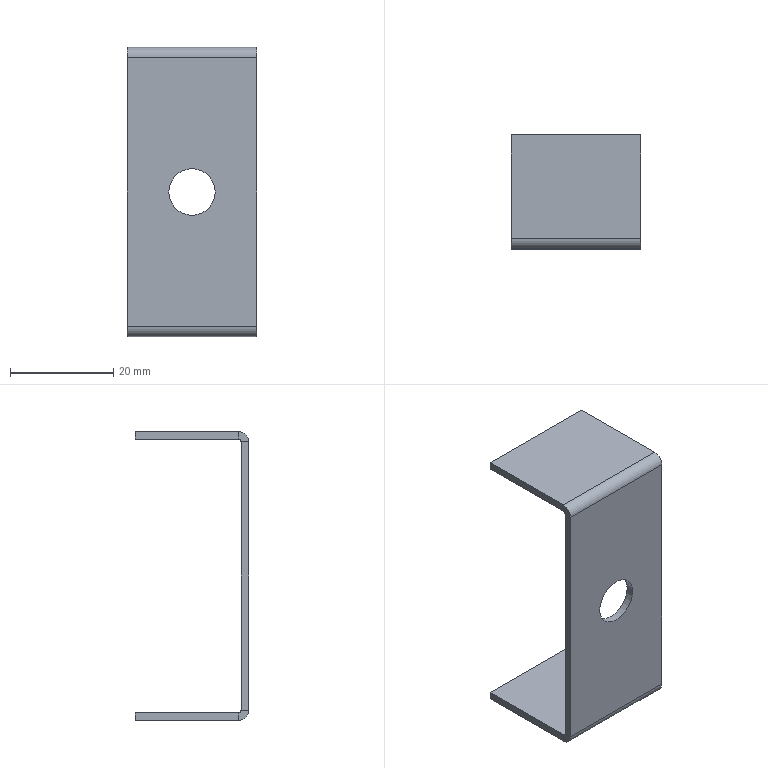Component | SolidWorks | BrowBracketAssembly3-1_BrowBracket-1 | 1 solid | 24 faces | box 25 x 22 x 56 mm | volume 3502 mm3 | plane 18 | cylinder 6 | commonest cylinder face diameters 9 x2 4 x2 1 x2
STEP:
#1=COLOUR_RGB('',0.7922,0.8196,0.9333);
#2=FILL_AREA_STYLE_COLOUR('',#1);
#3=FILL_AREA_STYLE('',(#2));
#4=SURFACE_STYLE_FILL_AREA(#3);
#5=SURFACE_SIDE_STYLE('',(#4));
#6=SURFACE_STYLE_USAGE(.BOTH.,#5);
#7=PRESENTATION_STYLE_ASSIGNMENT((#6));
#8=CARTESIAN_POINT('',(-2.047,6.292,1.181));
#9=VERTEX_POINT('',#8);
#10=CARTESIAN_POINT('',(-1.693,6.292,1.181));
#11=VERTEX_POINT('',#10);
#12=CARTESIAN_POINT('',(-1.87,6.292,1.181));
#13=DIRECTION('',(-0.,-1.,-0.));
#14=DIRECTION('',(1.,-0.,0.));
#15=AXIS2_PLACEMENT_3D('',#12,#13,#14);
#16=CIRCLE('',#15,0.1772);
#17=EDGE_CURVE('',#9,#11,#16,.T.);
#18=ORIENTED_EDGE('',*,*,#17,.F.);
#19=CARTESIAN_POINT('',(-2.047,6.233,1.181));
#20=VERTEX_POINT('',#19);
#21=CARTESIAN_POINT('',(-2.047,6.292,1.181));
#22=DIRECTION('',(-0.,-1.,-0.));
#23=VECTOR('',#22,39.37);
#24=LINE('',#21,#23);
#25=EDGE_CURVE('',#9,#20,#24,.T.);
#26=ORIENTED_EDGE('',*,*,#25,.T.);
#27=CARTESIAN_POINT('',(-1.693,6.233,1.181));
#28=VERTEX_POINT('',#27);
#29=CARTESIAN_POINT('',(-1.87,6.233,1.181));
#30=DIRECTION('',(-0.,-1.,-0.));
#31=DIRECTION('',(1.,-0.,0.));
#32=AXIS2_PLACEMENT_3D('',#29,#30,#31);
#33=CIRCLE('',#32,0.1772);
#34=EDGE_CURVE('',#20,#28,#33,.T.);
#35=ORIENTED_EDGE('',*,*,#34,.T.);
#36=CARTESIAN_POINT('',(-1.693,6.292,1.181));
#37=DIRECTION('',(-0.,-1.,-0.));
#38=VECTOR('',#37,39.37);
#39=LINE('',#36,#38);
#40=EDGE_CURVE('',#11,#28,#39,.T.);
#41=ORIENTED_EDGE('',*,*,#40,.F.);
#42=EDGE_LOOP('',(#18,#26,#35,#41));
#43=FACE_OUTER_BOUND('',#42,.T.);
#44=CARTESIAN_POINT('',(-1.87,6.292,1.181));
#45=DIRECTION('',(-0.,-1.,-0.));
#46=DIRECTION('',(1.,-0.,0.));
#47=AXIS2_PLACEMENT_3D('',#44,#45,#46);
#48=CYLINDRICAL_SURFACE('',#47,0.1772);
#49=ADVANCED_FACE('',(#43),#48,.F.);
#50=CARTESIAN_POINT('',(-2.362,6.233,2.204));
#51=VERTEX_POINT('',#50);
#52=CARTESIAN_POINT('',(-2.362,6.292,2.204));
#53=VERTEX_POINT('',#52);
#54=CARTESIAN_POINT('',(-2.362,6.233,2.204));
#55=DIRECTION('',(0.,1.,0.));
#56=VECTOR('',#55,39.37);
#57=LINE('',#54,#56);
#58=EDGE_CURVE('',#51,#53,#57,.T.);
#59=ORIENTED_EDGE('',*,*,#58,.F.);
#60=CARTESIAN_POINT('',(-2.362,6.311,2.283));
#61=VERTEX_POINT('',#60);
#62=CARTESIAN_POINT('',(-2.362,6.311,2.204));
#63=DIRECTION('',(1.,-0.,0.));
#64=DIRECTION('',(-0.,-1.,-0.));
#65=AXIS2_PLACEMENT_3D('',#62,#63,#64);
#66=CIRCLE('',#65,0.07874);
#67=EDGE_CURVE('',#61,#51,#66,.T.);
#68=ORIENTED_EDGE('',*,*,#67,.F.);
#69=CARTESIAN_POINT('',(-2.362,6.311,2.224));
#70=VERTEX_POINT('',#69);
#71=CARTESIAN_POINT('',(-2.362,6.311,2.224));
#72=DIRECTION('',(-0.,-0.,1.));
#73=VECTOR('',#72,39.37);
#74=LINE('',#71,#73);
#75=EDGE_CURVE('',#70,#61,#74,.T.);
#76=ORIENTED_EDGE('',*,*,#75,.F.);
#77=CARTESIAN_POINT('',(-2.362,6.311,2.204));
#78=DIRECTION('',(1.,-0.,0.));
#79=DIRECTION('',(-0.,-1.,-0.));
#80=AXIS2_PLACEMENT_3D('',#77,#78,#79);
#81=CIRCLE('',#80,0.01969);
#82=EDGE_CURVE('',#70,#53,#81,.T.);
#83=ORIENTED_EDGE('',*,*,#82,.T.);
#84=EDGE_LOOP('',(#59,#68,#76,#83));
#85=FACE_OUTER_BOUND('',#84,.T.);
#86=CARTESIAN_POINT('',(-2.362,6.233,2.204));
#87=DIRECTION('',(-1.,0.,-0.));
#88=DIRECTION('',(-0.,-1.,-0.));
#89=AXIS2_PLACEMENT_3D('',#86,#87,#88);
#90=PLANE('',#89);
#91=ADVANCED_FACE('',(#85),#90,.T.);
#92=CARTESIAN_POINT('',(-2.362,6.233,0.1571));
#93=VERTEX_POINT('',#92);
#94=CARTESIAN_POINT('',(-2.362,6.233,2.283));
#95=DIRECTION('',(0.,0.,-1.));
#96=VECTOR('',#95,39.37);
#97=LINE('',#94,#96);
#98=EDGE_CURVE('',#51,#93,#97,.T.);
#99=ORIENTED_EDGE('',*,*,#98,.F.);
#100=ORIENTED_EDGE('',*,*,#58,.T.);
#101=CARTESIAN_POINT('',(-2.362,6.292,0.1571));
#102=VERTEX_POINT('',#101);
#103=CARTESIAN_POINT('',(-2.362,6.292,2.283));
#104=DIRECTION('',(0.,0.,-1.));
#105=VECTOR('',#104,39.37);
#106=LINE('',#103,#105);
#107=EDGE_CURVE('',#53,#102,#106,.T.);
#108=ORIENTED_EDGE('',*,*,#107,.T.);
#109=CARTESIAN_POINT('',(-2.362,6.292,0.1571));
#110=DIRECTION('',(-0.,-1.,-0.));
#111=VECTOR('',#110,39.37);
#112=LINE('',#109,#111);
#113=EDGE_CURVE('',#102,#93,#112,.T.);
#114=ORIENTED_EDGE('',*,*,#113,.T.);
#115=EDGE_LOOP('',(#99,#100,#108,#114));
#116=FACE_OUTER_BOUND('',#115,.T.);
#117=CARTESIAN_POINT('',(-2.362,6.311,2.224));
#118=DIRECTION('',(-1.,0.,-0.));
#119=DIRECTION('',(-0.,-1.,-0.));
#120=AXIS2_PLACEMENT_3D('',#117,#118,#119);
#121=PLANE('',#120);
#122=ADVANCED_FACE('',(#116),#121,.T.);
#123=CARTESIAN_POINT('',(-1.378,6.311,2.283));
#124=VERTEX_POINT('',#123);
#125=CARTESIAN_POINT('',(-1.378,6.311,2.224));
#126=VERTEX_POINT('',#125);
#127=CARTESIAN_POINT('',(-1.378,6.311,2.283));
#128=DIRECTION('',(0.,0.,-1.));
#129=VECTOR('',#128,39.37);
#130=LINE('',#127,#129);
#131=EDGE_CURVE('',#124,#126,#130,.T.);
#132=ORIENTED_EDGE('',*,*,#131,.F.);
#133=CARTESIAN_POINT('',(-1.378,6.233,2.204));
#134=VERTEX_POINT('',#133);
#135=CARTESIAN_POINT('',(-1.378,6.311,2.204));
#136=DIRECTION('',(1.,-0.,0.));
#137=DIRECTION('',(-0.,-1.,-0.));
#138=AXIS2_PLACEMENT_3D('',#135,#136,#137);
#139=CIRCLE('',#138,0.07874);
#140=EDGE_CURVE('',#124,#134,#139,.T.);
#141=ORIENTED_EDGE('',*,*,#140,.T.);
#142=CARTESIAN_POINT('',(-1.378,6.292,2.204));
#143=VERTEX_POINT('',#142);
#144=CARTESIAN_POINT('',(-1.378,6.292,2.204));
#145=DIRECTION('',(-0.,-1.,-0.));
#146=VECTOR('',#145,39.37);
#147=LINE('',#144,#146);
#148=EDGE_CURVE('',#143,#134,#147,.T.);
#149=ORIENTED_EDGE('',*,*,#148,.F.);
#150=CARTESIAN_POINT('',(-1.378,6.311,2.204));
#151=DIRECTION('',(1.,-0.,0.));
#152=DIRECTION('',(-0.,-1.,0.));
#153=AXIS2_PLACEMENT_3D('',#150,#151,#152);
#154=CIRCLE('',#153,0.01969);
#155=EDGE_CURVE('',#126,#143,#154,.T.);
#156=ORIENTED_EDGE('',*,*,#155,.F.);
#157=EDGE_LOOP('',(#132,#141,#149,#156));
#158=FACE_OUTER_BOUND('',#157,.T.);
#159=CARTESIAN_POINT('',(-1.378,6.311,2.283));
#160=DIRECTION('',(1.,-0.,0.));
#161=DIRECTION('',(0.,1.,0.));
#162=AXIS2_PLACEMENT_3D('',#159,#160,#161);
#163=PLANE('',#162);
#164=ADVANCED_FACE('',(#158),#163,.T.);
#165=CARTESIAN_POINT('',(-1.378,7.099,2.283));
#166=VERTEX_POINT('',#165);
#167=CARTESIAN_POINT('',(-1.378,7.099,2.283));
#168=DIRECTION('',(-0.,-1.,-0.));
#169=VECTOR('',#168,39.37);
#170=LINE('',#167,#169);
#171=EDGE_CURVE('',#166,#124,#170,.T.);
#172=ORIENTED_EDGE('',*,*,#171,.T.);
#173=ORIENTED_EDGE('',*,*,#131,.T.);
#174=CARTESIAN_POINT('',(-1.378,7.099,2.224));
#175=VERTEX_POINT('',#174);
#176=CARTESIAN_POINT('',(-1.378,7.099,2.224));
#177=DIRECTION('',(-0.,-1.,-0.));
#178=VECTOR('',#177,39.37);
#179=LINE('',#176,#178);
#180=EDGE_CURVE('',#175,#126,#179,.T.);
#181=ORIENTED_EDGE('',*,*,#180,.F.);
#182=CARTESIAN_POINT('',(-1.378,7.099,2.224));
#183=DIRECTION('',(-0.,-0.,1.));
#184=VECTOR('',#183,39.37);
#185=LINE('',#182,#184);
#186=EDGE_CURVE('',#175,#166,#185,.T.);
#187=ORIENTED_EDGE('',*,*,#186,.T.);
#188=EDGE_LOOP('',(#172,#173,#181,#187));
#189=FACE_OUTER_BOUND('',#188,.T.);
#190=CARTESIAN_POINT('',(-1.378,6.292,2.204));
#191=DIRECTION('',(1.,-0.,0.));
#192=DIRECTION('',(0.,1.,0.));
#193=AXIS2_PLACEMENT_3D('',#190,#191,#192);
#194=PLANE('',#193);
#195=ADVANCED_FACE('',(#189),#194,.T.);
#196=CARTESIAN_POINT('',(-2.362,6.311,0.07841));
#197=VERTEX_POINT('',#196);
#198=CARTESIAN_POINT('',(-2.362,6.311,0.1375));
#199=VERTEX_POINT('',#198);
#200=CARTESIAN_POINT('',(-2.362,6.311,0.07841));
#201=DIRECTION('',(-0.,-0.,1.));
#202=VECTOR('',#201,39.37);
#203=LINE('',#200,#202);
#204=EDGE_CURVE('',#197,#199,#203,.T.);
#205=ORIENTED_EDGE('',*,*,#204,.F.);
#206=CARTESIAN_POINT('',(-2.362,6.311,0.1571));
#207=DIRECTION('',(1.,-0.,0.));
#208=DIRECTION('',(-0.,-1.,-0.));
#209=AXIS2_PLACEMENT_3D('',#206,#207,#208);
#210=CIRCLE('',#209,0.07874);
#211=EDGE_CURVE('',#93,#197,#210,.T.);
#212=ORIENTED_EDGE('',*,*,#211,.F.);
#213=ORIENTED_EDGE('',*,*,#113,.F.);
#214=CARTESIAN_POINT('',(-2.362,6.311,0.1571));
#215=DIRECTION('',(1.,-0.,0.));
#216=DIRECTION('',(-0.,-1.,-0.));
#217=AXIS2_PLACEMENT_3D('',#214,#215,#216);
#218=CIRCLE('',#217,0.01969);
#219=EDGE_CURVE('',#102,#199,#218,.T.);
#220=ORIENTED_EDGE('',*,*,#219,.T.);
#221=EDGE_LOOP('',(#205,#212,#213,#220));
#222=FACE_OUTER_BOUND('',#221,.T.);
#223=CARTESIAN_POINT('',(-2.362,6.311,0.07841));
#224=DIRECTION('',(-1.,0.,-0.));
#225=DIRECTION('',(-0.,-1.,-0.));
#226=AXIS2_PLACEMENT_3D('',#223,#224,#225);
#227=PLANE('',#226);
#228=ADVANCED_FACE('',(#222),#227,.T.);
#229=CARTESIAN_POINT('',(-2.362,7.099,0.07841));
#230=VERTEX_POINT('',#229);
#231=CARTESIAN_POINT('',(-2.362,6.233,0.07841));
#232=DIRECTION('',(0.,1.,0.));
#233=VECTOR('',#232,39.37);
#234=LINE('',#231,#233);
#235=EDGE_CURVE('',#197,#230,#234,.T.);
#236=ORIENTED_EDGE('',*,*,#235,.F.);
#237=ORIENTED_EDGE('',*,*,#204,.T.);
#238=CARTESIAN_POINT('',(-2.362,7.099,0.1375));
#239=VERTEX_POINT('',#238);
#240=CARTESIAN_POINT('',(-2.362,6.233,0.1375));
#241=DIRECTION('',(0.,1.,0.));
#242=VECTOR('',#241,39.37);
#243=LINE('',#240,#242);
#244=EDGE_CURVE('',#199,#239,#243,.T.);
#245=ORIENTED_EDGE('',*,*,#244,.T.);
#246=CARTESIAN_POINT('',(-2.362,7.099,0.07841));
#247=DIRECTION('',(-0.,-0.,1.));
#248=VECTOR('',#247,39.37);
#249=LINE('',#246,#248);
#250=EDGE_CURVE('',#230,#239,#249,.T.);
#251=ORIENTED_EDGE('',*,*,#250,.F.);
#252=EDGE_LOOP('',(#236,#237,#245,#251));
#253=FACE_OUTER_BOUND('',#252,.T.);
#254=CARTESIAN_POINT('',(-2.362,6.292,0.1571));
#255=DIRECTION('',(-1.,0.,-0.));
#256=DIRECTION('',(-0.,-1.,-0.));
#257=AXIS2_PLACEMENT_3D('',#254,#255,#256);
#258=PLANE('',#257);
#259=ADVANCED_FACE('',(#253),#258,.T.);
#260=CARTESIAN_POINT('',(-1.378,6.233,0.1571));
#261=VERTEX_POINT('',#260);
#262=CARTESIAN_POINT('',(-1.378,6.292,0.1571));
#263=VERTEX_POINT('',#262);
#264=CARTESIAN_POINT('',(-1.378,6.233,0.1571));
#265=DIRECTION('',(0.,1.,0.));
#266=VECTOR('',#265,39.37);
#267=LINE('',#264,#266);
#268=EDGE_CURVE('',#261,#263,#267,.T.);
#269=ORIENTED_EDGE('',*,*,#268,.F.);
#270=CARTESIAN_POINT('',(-1.378,6.311,0.07841));
#271=VERTEX_POINT('',#270);
#272=CARTESIAN_POINT('',(-1.378,6.311,0.1571));
#273=DIRECTION('',(1.,-0.,0.));
#274=DIRECTION('',(-0.,-1.,-0.));
#275=AXIS2_PLACEMENT_3D('',#272,#273,#274);
#276=CIRCLE('',#275,0.07874);
#277=EDGE_CURVE('',#261,#271,#276,.T.);
#278=ORIENTED_EDGE('',*,*,#277,.T.);
#279=CARTESIAN_POINT('',(-1.378,6.311,0.1375));
#280=VERTEX_POINT('',#279);
#281=CARTESIAN_POINT('',(-1.378,6.311,0.1375));
#282=DIRECTION('',(0.,0.,-1.));
#283=VECTOR('',#282,39.37);
#284=LINE('',#281,#283);
#285=EDGE_CURVE('',#280,#271,#284,.T.);
#286=ORIENTED_EDGE('',*,*,#285,.F.);
#287=CARTESIAN_POINT('',(-1.378,6.311,0.1571));
#288=DIRECTION('',(1.,-0.,0.));
#289=DIRECTION('',(-0.,-1.,-0.));
#290=AXIS2_PLACEMENT_3D('',#287,#288,#289);
#291=CIRCLE('',#290,0.01969);
#292=EDGE_CURVE('',#263,#280,#291,.T.);
#293=ORIENTED_EDGE('',*,*,#292,.F.);
#294=EDGE_LOOP('',(#269,#278,#286,#293));
#295=FACE_OUTER_BOUND('',#294,.T.);
#296=CARTESIAN_POINT('',(-1.378,6.233,0.1571));
#297=DIRECTION('',(1.,-0.,0.));
#298=DIRECTION('',(0.,1.,0.));
#299=AXIS2_PLACEMENT_3D('',#296,#297,#298);
#300=PLANE('',#299);
#301=ADVANCED_FACE('',(#295),#300,.T.);
#302=CARTESIAN_POINT('',(-1.378,6.233,2.283));
#303=DIRECTION('',(0.,0.,-1.));
#304=VECTOR('',#303,39.37);
#305=LINE('',#302,#304);
#306=EDGE_CURVE('',#134,#261,#305,.T.);
#307=ORIENTED_EDGE('',*,*,#306,.T.);
#308=ORIENTED_EDGE('',*,*,#268,.T.);
#309=CARTESIAN_POINT('',(-1.378,6.292,2.283));
#310=DIRECTION('',(0.,0.,-1.));
#311=VECTOR('',#310,39.37);
#312=LINE('',#309,#311);
#313=EDGE_CURVE('',#143,#263,#312,.T.);
#314=ORIENTED_EDGE('',*,*,#313,.F.);
#315=ORIENTED_EDGE('',*,*,#148,.T.);
#316=EDGE_LOOP('',(#307,#308,#314,#315));
#317=FACE_OUTER_BOUND('',#316,.T.);
#318=CARTESIAN_POINT('',(-1.378,6.311,0.1375));
#319=DIRECTION('',(1.,-0.,0.));
#320=DIRECTION('',(0.,1.,0.));
#321=AXIS2_PLACEMENT_3D('',#318,#319,#320);
#322=PLANE('',#321);
#323=ADVANCED_FACE('',(#317),#322,.T.);
#324=CARTESIAN_POINT('',(-1.378,7.099,0.1375));
#325=VERTEX_POINT('',#324);
#326=CARTESIAN_POINT('',(-1.378,6.233,0.1375));
#327=DIRECTION('',(0.,1.,0.));
#328=VECTOR('',#327,39.37);
#329=LINE('',#326,#328);
#330=EDGE_CURVE('',#280,#325,#329,.T.);
#331=ORIENTED_EDGE('',*,*,#330,.T.);
#332=CARTESIAN_POINT('',(-2.362,7.099,0.1375));
#333=DIRECTION('',(1.,-0.,0.));
#334=VECTOR('',#333,39.37);
#335=LINE('',#332,#334);
#336=EDGE_CURVE('',#239,#325,#335,.T.);
#337=ORIENTED_EDGE('',*,*,#336,.F.);
#338=ORIENTED_EDGE('',*,*,#244,.F.);
#339=CARTESIAN_POINT('',(-2.362,6.311,0.1375));
#340=DIRECTION('',(1.,-0.,0.));
#341=VECTOR('',#340,39.37);
#342=LINE('',#339,#341);
#343=EDGE_CURVE('',#199,#280,#342,.T.);
#344=ORIENTED_EDGE('',*,*,#343,.T.);
#345=EDGE_LOOP('',(#331,#337,#338,#344));
#346=FACE_OUTER_BOUND('',#345,.T.);
#347=CARTESIAN_POINT('',(-2.362,6.233,0.1375));
#348=DIRECTION('',(0.,0.,-1.));
#349=DIRECTION('',(-0.,-1.,-0.));
#350=AXIS2_PLACEMENT_3D('',#347,#348,#349);
#351=PLANE('',#350);
#352=ADVANCED_FACE('',(#346),#351,.F.);
#353=CARTESIAN_POINT('',(-1.378,7.099,0.07841));
#354=VERTEX_POINT('',#353);
#355=CARTESIAN_POINT('',(-1.378,7.099,0.07841));
#356=DIRECTION('',(-0.,-0.,1.));
#357=VECTOR('',#356,39.37);
#358=LINE('',#355,#357);
#359=EDGE_CURVE('',#354,#325,#358,.T.);
#360=ORIENTED_EDGE('',*,*,#359,.F.);
#361=CARTESIAN_POINT('',(-2.362,7.099,0.07841));
#362=DIRECTION('',(1.,-0.,0.));
#363=VECTOR('',#362,39.37);
#364=LINE('',#361,#363);
#365=EDGE_CURVE('',#230,#354,#364,.T.);
#366=ORIENTED_EDGE('',*,*,#365,.F.);
#367=ORIENTED_EDGE('',*,*,#250,.T.);
#368=ORIENTED_EDGE('',*,*,#336,.T.);
#369=EDGE_LOOP('',(#360,#366,#367,#368));
#370=FACE_OUTER_BOUND('',#369,.T.);
#371=CARTESIAN_POINT('',(-2.362,7.099,0.07841));
#372=DIRECTION('',(0.,1.,0.));
#373=DIRECTION('',(-1.,0.,-0.));
#374=AXIS2_PLACEMENT_3D('',#371,#372,#373);
#375=PLANE('',#374);
#376=ADVANCED_FACE('',(#370),#375,.T.);
#377=CARTESIAN_POINT('',(-1.378,6.233,0.07841));
#378=DIRECTION('',(0.,1.,0.));
#379=VECTOR('',#378,39.37);
#380=LINE('',#377,#379);
#381=EDGE_CURVE('',#271,#354,#380,.T.);
#382=ORIENTED_EDGE('',*,*,#381,.F.);
#383=CARTESIAN_POINT('',(-2.362,6.311,0.07841));
#384=DIRECTION('',(1.,-0.,0.));
#385=VECTOR('',#384,39.37);
#386=LINE('',#383,#385);
#387=EDGE_CURVE('',#197,#271,#386,.T.);
#388=ORIENTED_EDGE('',*,*,#387,.F.);
#389=ORIENTED_EDGE('',*,*,#235,.T.);
#390=ORIENTED_EDGE('',*,*,#365,.T.);
#391=EDGE_LOOP('',(#382,#388,#389,#390));
#392=FACE_OUTER_BOUND('',#391,.T.);
#393=CARTESIAN_POINT('',(-2.362,6.233,0.07841));
#394=DIRECTION('',(0.,0.,-1.));
#395=DIRECTION('',(-0.,-1.,-0.));
#396=AXIS2_PLACEMENT_3D('',#393,#394,#395);
#397=PLANE('',#396);
#398=ADVANCED_FACE('',(#392),#397,.T.);
#399=ORIENTED_EDGE('',*,*,#277,.F.);
#400=CARTESIAN_POINT('',(-2.362,6.233,0.1571));
#401=DIRECTION('',(1.,-0.,0.));
#402=VECTOR('',#401,39.37);
#403=LINE('',#400,#402);
#404=EDGE_CURVE('',#93,#261,#403,.T.);
#405=ORIENTED_EDGE('',*,*,#404,.F.);
#406=ORIENTED_EDGE('',*,*,#211,.T.);
#407=ORIENTED_EDGE('',*,*,#387,.T.);
#408=EDGE_LOOP('',(#399,#405,#406,#407));
#409=FACE_OUTER_BOUND('',#408,.T.);
#410=CARTESIAN_POINT('',(-2.362,6.311,0.1571));
#411=DIRECTION('',(1.,-0.,0.));
#412=DIRECTION('',(0.,1.,0.));
#413=AXIS2_PLACEMENT_3D('',#410,#411,#412);
#414=CYLINDRICAL_SURFACE('',#413,0.07874);
#415=ADVANCED_FACE('',(#409),#414,.T.);
#416=CARTESIAN_POINT('',(-1.87,6.233,1.181));
#417=DIRECTION('',(-0.,-1.,-0.));
#418=DIRECTION('',(1.,-0.,0.));
#419=AXIS2_PLACEMENT_3D('',#416,#417,#418);
#420=CIRCLE('',#419,0.1772);
#421=EDGE_CURVE('',#28,#20,#420,.T.);
#422=ORIENTED_EDGE('',*,*,#421,.F.);
#423=ORIENTED_EDGE('',*,*,#34,.F.);
#424=EDGE_LOOP('',(#422,#423));
#425=FACE_BOUND('',#424,.T.);
#426=ORIENTED_EDGE('',*,*,#306,.F.);
#427=CARTESIAN_POINT('',(-2.362,6.233,2.204));
#428=DIRECTION('',(1.,-0.,0.));
#429=VECTOR('',#428,39.37);
#430=LINE('',#427,#429);
#431=EDGE_CURVE('',#51,#134,#430,.T.);
#432=ORIENTED_EDGE('',*,*,#431,.F.);
#433=ORIENTED_EDGE('',*,*,#98,.T.);
#434=ORIENTED_EDGE('',*,*,#404,.T.);
#435=EDGE_LOOP('',(#426,#432,#433,#434));
#436=FACE_OUTER_BOUND('',#435,.T.);
#437=CARTESIAN_POINT('',(-2.362,6.233,2.283));
#438=DIRECTION('',(-0.,-1.,-0.));
#439=DIRECTION('',(1.,-0.,0.));
#440=AXIS2_PLACEMENT_3D('',#437,#438,#439);
#441=PLANE('',#440);
#442=ADVANCED_FACE('',(#425,#436),#441,.T.);
#443=ORIENTED_EDGE('',*,*,#140,.F.);
#444=CARTESIAN_POINT('',(-2.362,6.311,2.283));
#445=DIRECTION('',(1.,-0.,0.));
#446=VECTOR('',#445,39.37);
#447=LINE('',#444,#446);
#448=EDGE_CURVE('',#61,#124,#447,.T.);
#449=ORIENTED_EDGE('',*,*,#448,.F.);
#450=ORIENTED_EDGE('',*,*,#67,.T.);
#451=ORIENTED_EDGE('',*,*,#431,.T.);
#452=EDGE_LOOP('',(#443,#449,#450,#451));
#453=FACE_OUTER_BOUND('',#452,.T.);
#454=CARTESIAN_POINT('',(-2.362,6.311,2.204));
#455=DIRECTION('',(1.,-0.,0.));
#456=DIRECTION('',(0.,1.,0.));
#457=AXIS2_PLACEMENT_3D('',#454,#455,#456);
#458=CYLINDRICAL_SURFACE('',#457,0.07874);
#459=ADVANCED_FACE('',(#453),#458,.T.);
#460=ORIENTED_EDGE('',*,*,#171,.F.);
#461=CARTESIAN_POINT('',(-2.362,7.099,2.283));
#462=VERTEX_POINT('',#461);
#463=CARTESIAN_POINT('',(-2.362,7.099,2.283));
#464=DIRECTION('',(1.,-0.,0.));
#465=VECTOR('',#464,39.37);
#466=LINE('',#463,#465);
#467=EDGE_CURVE('',#462,#166,#466,.T.);
#468=ORIENTED_EDGE('',*,*,#467,.F.);
#469=CARTESIAN_POINT('',(-2.362,7.099,2.283));
#470=DIRECTION('',(-0.,-1.,-0.));
#471=VECTOR('',#470,39.37);
#472=LINE('',#469,#471);
#473=EDGE_CURVE('',#462,#61,#472,.T.);
#474=ORIENTED_EDGE('',*,*,#473,.T.);
#475=ORIENTED_EDGE('',*,*,#448,.T.);
#476=EDGE_LOOP('',(#460,#468,#474,#475));
#477=FACE_OUTER_BOUND('',#476,.T.);
#478=CARTESIAN_POINT('',(-2.362,7.099,2.283));
#479=DIRECTION('',(-0.,-0.,1.));
#480=DIRECTION('',(-1.,0.,-0.));
#481=AXIS2_PLACEMENT_3D('',#478,#479,#480);
#482=PLANE('',#481);
#483=ADVANCED_FACE('',(#477),#482,.T.);
#484=ORIENTED_EDGE('',*,*,#186,.F.);
#485=CARTESIAN_POINT('',(-2.362,7.099,2.224));
#486=VERTEX_POINT('',#485);
#487=CARTESIAN_POINT('',(-2.362,7.099,2.224));
#488=DIRECTION('',(1.,-0.,0.));
#489=VECTOR('',#488,39.37);
#490=LINE('',#487,#489);
#491=EDGE_CURVE('',#486,#175,#490,.T.);
#492=ORIENTED_EDGE('',*,*,#491,.F.);
#493=CARTESIAN_POINT('',(-2.362,7.099,2.224));
#494=DIRECTION('',(-0.,-0.,1.));
#495=VECTOR('',#494,39.37);
#496=LINE('',#493,#495);
#497=EDGE_CURVE('',#486,#462,#496,.T.);
#498=ORIENTED_EDGE('',*,*,#497,.T.);
#499=ORIENTED_EDGE('',*,*,#467,.T.);
#500=EDGE_LOOP('',(#484,#492,#498,#499));
#501=FACE_OUTER_BOUND('',#500,.T.);
#502=CARTESIAN_POINT('',(-2.362,7.099,2.224));
#503=DIRECTION('',(0.,1.,0.));
#504=DIRECTION('',(-1.,0.,-0.));
#505=AXIS2_PLACEMENT_3D('',#502,#503,#504);
#506=PLANE('',#505);
#507=ADVANCED_FACE('',(#501),#506,.T.);
#508=ORIENTED_EDGE('',*,*,#180,.T.);
#509=CARTESIAN_POINT('',(-2.362,6.311,2.224));
#510=DIRECTION('',(1.,-0.,0.));
#511=VECTOR('',#510,39.37);
#512=LINE('',#509,#511);
#513=EDGE_CURVE('',#70,#126,#512,.T.);
#514=ORIENTED_EDGE('',*,*,#513,.F.);
#515=CARTESIAN_POINT('',(-2.362,7.099,2.224));
#516=DIRECTION('',(-0.,-1.,-0.));
#517=VECTOR('',#516,39.37);
#518=LINE('',#515,#517);
#519=EDGE_CURVE('',#486,#70,#518,.T.);
#520=ORIENTED_EDGE('',*,*,#519,.F.);
#521=ORIENTED_EDGE('',*,*,#491,.T.);
#522=EDGE_LOOP('',(#508,#514,#520,#521));
#523=FACE_OUTER_BOUND('',#522,.T.);
#524=CARTESIAN_POINT('',(-2.362,7.099,2.224));
#525=DIRECTION('',(-0.,-0.,1.));
#526=DIRECTION('',(-1.,0.,-0.));
#527=AXIS2_PLACEMENT_3D('',#524,#525,#526);
#528=PLANE('',#527);
#529=ADVANCED_FACE('',(#523),#528,.F.);
#530=ORIENTED_EDGE('',*,*,#155,.T.);
#531=CARTESIAN_POINT('',(-2.362,6.292,2.204));
#532=DIRECTION('',(1.,-0.,0.));
#533=VECTOR('',#532,39.37);
#534=LINE('',#531,#533);
#535=EDGE_CURVE('',#53,#143,#534,.T.);
#536=ORIENTED_EDGE('',*,*,#535,.F.);
#537=ORIENTED_EDGE('',*,*,#82,.F.);
#538=ORIENTED_EDGE('',*,*,#513,.T.);
#539=EDGE_LOOP('',(#530,#536,#537,#538));
#540=FACE_OUTER_BOUND('',#539,.T.);
#541=CARTESIAN_POINT('',(-2.362,6.311,2.204));
#542=DIRECTION('',(1.,-0.,0.));
#543=DIRECTION('',(0.,1.,0.));
#544=AXIS2_PLACEMENT_3D('',#541,#542,#543);
#545=CYLINDRICAL_SURFACE('',#544,0.01969);
#546=ADVANCED_FACE('',(#540),#545,.F.);
#547=CARTESIAN_POINT('',(-1.87,6.292,1.181));
#548=DIRECTION('',(-0.,-1.,-0.));
#549=DIRECTION('',(1.,-0.,0.));
#550=AXIS2_PLACEMENT_3D('',#547,#548,#549);
#551=CIRCLE('',#550,0.1772);
#552=EDGE_CURVE('',#11,#9,#551,.T.);
#553=ORIENTED_EDGE('',*,*,#552,.T.);
#554=ORIENTED_EDGE('',*,*,#17,.T.);
#555=EDGE_LOOP('',(#553,#554));
#556=FACE_BOUND('',#555,.T.);
#557=ORIENTED_EDGE('',*,*,#313,.T.);
#558=CARTESIAN_POINT('',(-2.362,6.292,0.1571));
#559=DIRECTION('',(1.,-0.,0.));
#560=VECTOR('',#559,39.37);
#561=LINE('',#558,#560);
#562=EDGE_CURVE('',#102,#263,#561,.T.);
#563=ORIENTED_EDGE('',*,*,#562,.F.);
#564=ORIENTED_EDGE('',*,*,#107,.F.);
#565=ORIENTED_EDGE('',*,*,#535,.T.);
#566=EDGE_LOOP('',(#557,#563,#564,#565));
#567=FACE_OUTER_BOUND('',#566,.T.);
#568=CARTESIAN_POINT('',(-2.362,6.292,2.283));
#569=DIRECTION('',(-0.,-1.,-0.));
#570=DIRECTION('',(1.,-0.,0.));
#571=AXIS2_PLACEMENT_3D('',#568,#569,#570);
#572=PLANE('',#571);
#573=ADVANCED_FACE('',(#556,#567),#572,.F.);
#574=ORIENTED_EDGE('',*,*,#292,.T.);
#575=ORIENTED_EDGE('',*,*,#343,.F.);
#576=ORIENTED_EDGE('',*,*,#219,.F.);
#577=ORIENTED_EDGE('',*,*,#562,.T.);
#578=EDGE_LOOP('',(#574,#575,#576,#577));
#579=FACE_OUTER_BOUND('',#578,.T.);
#580=CARTESIAN_POINT('',(-2.362,6.311,0.1571));
#581=DIRECTION('',(1.,-0.,0.));
#582=DIRECTION('',(0.,1.,0.));
#583=AXIS2_PLACEMENT_3D('',#580,#581,#582);
#584=CYLINDRICAL_SURFACE('',#583,0.01969);
#585=ADVANCED_FACE('',(#579),#584,.F.);
#586=ORIENTED_EDGE('',*,*,#519,.T.);
#587=ORIENTED_EDGE('',*,*,#75,.T.);
#588=ORIENTED_EDGE('',*,*,#473,.F.);
#589=ORIENTED_EDGE('',*,*,#497,.F.);
#590=EDGE_LOOP('',(#586,#587,#588,#589));
#591=FACE_OUTER_BOUND('',#590,.T.);
#592=CARTESIAN_POINT('',(-2.362,6.311,0.1571));
#593=DIRECTION('',(-1.,0.,-0.));
#594=DIRECTION('',(-0.,-1.,-0.));
#595=AXIS2_PLACEMENT_3D('',#592,#593,#594);
#596=PLANE('',#595);
#597=ADVANCED_FACE('',(#591),#596,.T.);
#598=ORIENTED_EDGE('',*,*,#330,.F.);
#599=ORIENTED_EDGE('',*,*,#285,.T.);
#600=ORIENTED_EDGE('',*,*,#381,.T.);
#601=ORIENTED_EDGE('',*,*,#359,.T.);
#602=EDGE_LOOP('',(#598,#599,#600,#601));
#603=FACE_OUTER_BOUND('',#602,.T.);
#604=CARTESIAN_POINT('',(-1.378,6.311,0.1571));
#605=DIRECTION('',(-1.,0.,-0.));
#606=DIRECTION('',(-0.,-1.,-0.));
#607=AXIS2_PLACEMENT_3D('',#604,#605,#606);
#608=PLANE('',#607);
#609=ADVANCED_FACE('',(#603),#608,.F.);
#610=ORIENTED_EDGE('',*,*,#25,.F.);
#611=ORIENTED_EDGE('',*,*,#552,.F.);
#612=ORIENTED_EDGE('',*,*,#40,.T.);
#613=ORIENTED_EDGE('',*,*,#421,.T.);
#614=EDGE_LOOP('',(#610,#611,#612,#613));
#615=FACE_OUTER_BOUND('',#614,.T.);
#616=CARTESIAN_POINT('',(-1.87,6.292,1.181));
#617=DIRECTION('',(-0.,-1.,-0.));
#618=DIRECTION('',(1.,-0.,0.));
#619=AXIS2_PLACEMENT_3D('',#616,#617,#618);
#620=CYLINDRICAL_SURFACE('',#619,0.1772);
#621=ADVANCED_FACE('',(#615),#620,.F.);
#622=CLOSED_SHELL('',(#49,#91,#122,#164,#195,#228,#259,#301,#323,#352,#376,#398,#415,#442,#459,#483,#507,#529,#546,#573,#585,#597,#609,#621));
#623=MANIFOLD_SOLID_BREP('',#622);
#624=STYLED_ITEM('',(#7),#623);
#625=(LENGTH_UNIT()NAMED_UNIT(*)SI_UNIT($,.METRE.));
#626=LENGTH_MEASURE_WITH_UNIT(LENGTH_MEASURE(0.0254),#625);
#627=DIMENSIONAL_EXPONENTS(1.,0.,0.,0.,0.,0.,0.);
#628=(CONVERSION_BASED_UNIT('',#626)LENGTH_UNIT()NAMED_UNIT(#627));
#629=UNCERTAINTY_MEASURE_WITH_UNIT(LENGTH_MEASURE(0.00001),#628,'','');
#630=(NAMED_UNIT(*)PLANE_ANGLE_UNIT()SI_UNIT($,.RADIAN.));
#631=(NAMED_UNIT(*)SI_UNIT($,.STERADIAN.)SOLID_ANGLE_UNIT());
#632=(GEOMETRIC_REPRESENTATION_CONTEXT(3)GLOBAL_UNCERTAINTY_ASSIGNED_CONTEXT((#629))GLOBAL_UNIT_ASSIGNED_CONTEXT((#628,#630,#631))REPRESENTATION_CONTEXT('',''));
#633=MECHANICAL_DESIGN_GEOMETRIC_PRESENTATION_REPRESENTATION('',(#624),#632);
#634=CARTESIAN_POINT('',(0.,0.,0.));
#635=DIRECTION('',(0.,0.,1.));
#636=DIRECTION('',(1.,0.,0.));
#637=AXIS2_PLACEMENT_3D('',#634,#635,#636);
#638=(LENGTH_UNIT()NAMED_UNIT(*)SI_UNIT($,.METRE.));
#639=LENGTH_MEASURE_WITH_UNIT(LENGTH_MEASURE(0.0254),#638);
#640=DIMENSIONAL_EXPONENTS(1.,0.,0.,0.,0.,0.,0.);
#641=(CONVERSION_BASED_UNIT('',#639)LENGTH_UNIT()NAMED_UNIT(#640));
#642=UNCERTAINTY_MEASURE_WITH_UNIT(LENGTH_MEASURE(0.00001),#641,'','');
#643=(NAMED_UNIT(*)PLANE_ANGLE_UNIT()SI_UNIT($,.RADIAN.));
#644=(NAMED_UNIT(*)SI_UNIT($,.STERADIAN.)SOLID_ANGLE_UNIT());
#645=(GEOMETRIC_REPRESENTATION_CONTEXT(3)GLOBAL_UNCERTAINTY_ASSIGNED_CONTEXT((#642))GLOBAL_UNIT_ASSIGNED_CONTEXT((#641,#643,#644))REPRESENTATION_CONTEXT('',''));
#646=ADVANCED_BREP_SHAPE_REPRESENTATION('',(#623,#637),#645);
#647=PRESENTATION_LAYER_ASSIGNMENT('','',(#624));